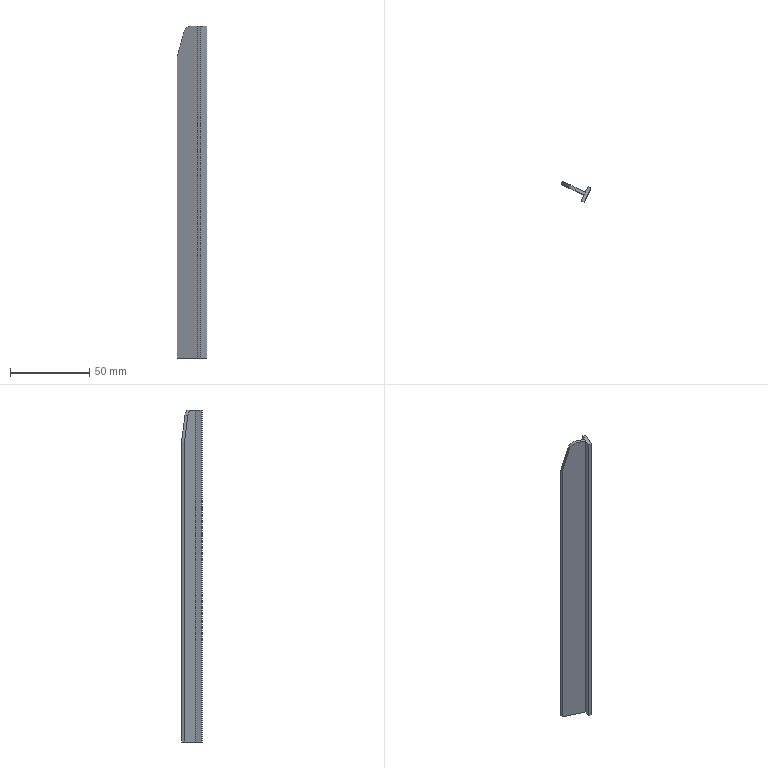Component | SolidWorks | JYTBJ-HeaderPlateClampBlock-1 | 1 solid | 12 faces | box 18.84 x 13.08 x 209 mm | volume 10743 mm3 | plane 11 | cylinder 1 | commonest cylinder face diameters 10 x1
build123d program:
from build123d import *

# Parameters (mm, degrees)
BOSS_EXTRUDE1_DEPTH = 209
CUT_EXTRUDE1_DEPTH  = 146
FILLET1_R           = 5


with BuildPart() as part:
    # Sketch1 → Boss-Extrude1 (new body)
    with BuildSketch(Plane.XY):
        Polygon((-5, 0), (5, 0), (5, 2), (1, 2), (1, 18), (-1, 18), (-1, 2), (-5, 2), align=None)
    extrude(amount=BOSS_EXTRUDE1_DEPTH)

    # Sketch3 → Cut-Extrude1 (cut)
    with BuildSketch(Plane(origin=(1, 0, 0), x_dir=(0, 0, -1), z_dir=(1, 0, 0))):
        Polygon((-20, 18), (0, 12), (0, 18), align=None)
    extrude(amount=-CUT_EXTRUDE1_DEPTH, mode=Mode.SUBTRACT)

    # Fillet1
    fillet1_edges = [part.edges().sort_by_distance(p)[0] for p in [
        (0, 12, 0),
    ]]
    fillet(fillet1_edges, radius=FILLET1_R)


solid = part.part

# Placed as in the assembly
solid = solid.moved(Location((-18.355, 107.069, 257.5), (-180, 0, 115.128)))
STEP:
#1=COLOUR_RGB('',0.7922,0.8196,0.9333);
#2=FILL_AREA_STYLE_COLOUR('',#1);
#3=FILL_AREA_STYLE('',(#2));
#4=SURFACE_STYLE_FILL_AREA(#3);
#5=SURFACE_SIDE_STYLE('',(#4));
#6=SURFACE_STYLE_USAGE(.BOTH.,#5);
#7=PRESENTATION_STYLE_ASSIGNMENT((#6));
#8=CARTESIAN_POINT('',(-1.348,4.552,9.35));
#9=VERTEX_POINT('',#8);
#10=CARTESIAN_POINT('',(-1.172,4.469,9.998));
#11=VERTEX_POINT('',#10);
#12=CARTESIAN_POINT('',(-3.155,5.399,2.697));
#13=DIRECTION('',(0.2602,-0.122,0.9578));
#14=VECTOR('',#13,39.37);
#15=LINE('',#12,#14);
#16=EDGE_CURVE('',#9,#11,#15,.T.);
#17=ORIENTED_EDGE('',*,*,#16,.T.);
#18=CARTESIAN_POINT('',(-1.001,4.389,10.138));
#19=VERTEX_POINT('',#18);
#20=CARTESIAN_POINT('',(-1.001,4.389,9.941));
#21=DIRECTION('',(0.4246,0.9054,0.));
#22=DIRECTION('',(0.,0.,1.));
#23=AXIS2_PLACEMENT_3D('',#20,#21,#22);
#24=CIRCLE('',#23,0.1969);
#25=EDGE_CURVE('',#11,#19,#24,.T.);
#26=ORIENTED_EDGE('',*,*,#25,.T.);
#27=CARTESIAN_POINT('',(-0.7772,4.284,10.138));
#28=VERTEX_POINT('',#27);
#29=CARTESIAN_POINT('',(-0.7772,4.284,10.138));
#30=DIRECTION('',(0.9054,-0.4246,0.));
#31=VECTOR('',#30,39.37);
#32=LINE('',#29,#31);
#33=EDGE_CURVE('',#19,#28,#32,.T.);
#34=ORIENTED_EDGE('',*,*,#33,.T.);
#35=CARTESIAN_POINT('',(-0.7772,4.284,1.909));
#36=VERTEX_POINT('',#35);
#37=CARTESIAN_POINT('',(-0.7772,4.284,1.909));
#38=DIRECTION('',(-0.,-0.,1.));
#39=VECTOR('',#38,39.37);
#40=LINE('',#37,#39);
#41=EDGE_CURVE('',#36,#28,#40,.T.);
#42=ORIENTED_EDGE('',*,*,#41,.F.);
#43=CARTESIAN_POINT('',(-1.348,4.552,1.909));
#44=VERTEX_POINT('',#43);
#45=CARTESIAN_POINT('',(-0.7772,4.284,1.909));
#46=DIRECTION('',(0.9054,-0.4246,0.));
#47=VECTOR('',#46,39.37);
#48=LINE('',#45,#47);
#49=EDGE_CURVE('',#44,#36,#48,.T.);
#50=ORIENTED_EDGE('',*,*,#49,.F.);
#51=CARTESIAN_POINT('',(-1.348,4.552,1.909));
#52=DIRECTION('',(-0.,-0.,1.));
#53=VECTOR('',#52,39.37);
#54=LINE('',#51,#53);
#55=EDGE_CURVE('',#44,#9,#54,.T.);
#56=ORIENTED_EDGE('',*,*,#55,.T.);
#57=EDGE_LOOP('',(#17,#26,#34,#42,#50,#56));
#58=FACE_OUTER_BOUND('',#57,.T.);
#59=CARTESIAN_POINT('',(-0.7772,4.284,1.909));
#60=DIRECTION('',(-0.4246,-0.9054,-0.));
#61=DIRECTION('',(-0.,-0.,1.));
#62=AXIS2_PLACEMENT_3D('',#59,#60,#61);
#63=PLANE('',#62);
#64=ADVANCED_FACE('',(#58),#63,.F.);
#65=CARTESIAN_POINT('',(-0.7104,4.427,10.138));
#66=VERTEX_POINT('',#65);
#67=CARTESIAN_POINT('',(-0.7104,4.427,10.138));
#68=DIRECTION('',(0.4246,0.9054,0.));
#69=VECTOR('',#68,39.37);
#70=LINE('',#67,#69);
#71=EDGE_CURVE('',#28,#66,#70,.T.);
#72=ORIENTED_EDGE('',*,*,#71,.T.);
#73=CARTESIAN_POINT('',(-0.7104,4.427,1.909));
#74=VERTEX_POINT('',#73);
#75=CARTESIAN_POINT('',(-0.7104,4.427,1.909));
#76=DIRECTION('',(-0.,-0.,1.));
#77=VECTOR('',#76,39.37);
#78=LINE('',#75,#77);
#79=EDGE_CURVE('',#74,#66,#78,.T.);
#80=ORIENTED_EDGE('',*,*,#79,.F.);
#81=CARTESIAN_POINT('',(-0.7104,4.427,1.909));
#82=DIRECTION('',(0.4246,0.9054,0.));
#83=VECTOR('',#82,39.37);
#84=LINE('',#81,#83);
#85=EDGE_CURVE('',#36,#74,#84,.T.);
#86=ORIENTED_EDGE('',*,*,#85,.F.);
#87=ORIENTED_EDGE('',*,*,#41,.T.);
#88=EDGE_LOOP('',(#72,#80,#86,#87));
#89=FACE_OUTER_BOUND('',#88,.T.);
#90=CARTESIAN_POINT('',(-0.7104,4.427,1.909));
#91=DIRECTION('',(0.9054,-0.4246,0.));
#92=DIRECTION('',(-0.4246,-0.9054,-0.));
#93=AXIS2_PLACEMENT_3D('',#90,#91,#92);
#94=PLANE('',#93);
#95=ADVANCED_FACE('',(#89),#94,.F.);
#96=CARTESIAN_POINT('',(-0.6391,4.394,10.138));
#97=VERTEX_POINT('',#96);
#98=CARTESIAN_POINT('',(-0.6391,4.394,10.138));
#99=DIRECTION('',(0.9054,-0.4246,0.));
#100=VECTOR('',#99,39.37);
#101=LINE('',#98,#100);
#102=EDGE_CURVE('',#66,#97,#101,.T.);
#103=ORIENTED_EDGE('',*,*,#102,.T.);
#104=CARTESIAN_POINT('',(-0.6391,4.394,1.909));
#105=VERTEX_POINT('',#104);
#106=CARTESIAN_POINT('',(-0.6391,4.394,1.909));
#107=DIRECTION('',(-0.,-0.,1.));
#108=VECTOR('',#107,39.37);
#109=LINE('',#106,#108);
#110=EDGE_CURVE('',#105,#97,#109,.T.);
#111=ORIENTED_EDGE('',*,*,#110,.F.);
#112=CARTESIAN_POINT('',(-0.6391,4.394,1.909));
#113=DIRECTION('',(0.9054,-0.4246,0.));
#114=VECTOR('',#113,39.37);
#115=LINE('',#112,#114);
#116=EDGE_CURVE('',#74,#105,#115,.T.);
#117=ORIENTED_EDGE('',*,*,#116,.F.);
#118=ORIENTED_EDGE('',*,*,#79,.T.);
#119=EDGE_LOOP('',(#103,#111,#117,#118));
#120=FACE_OUTER_BOUND('',#119,.T.);
#121=CARTESIAN_POINT('',(-0.6391,4.394,1.909));
#122=DIRECTION('',(-0.4246,-0.9054,-0.));
#123=DIRECTION('',(-0.,-0.,1.));
#124=AXIS2_PLACEMENT_3D('',#121,#122,#123);
#125=PLANE('',#124);
#126=ADVANCED_FACE('',(#120),#125,.F.);
#127=CARTESIAN_POINT('',(-0.8062,4.037,10.138));
#128=VERTEX_POINT('',#127);
#129=CARTESIAN_POINT('',(-0.6391,4.394,10.138));
#130=DIRECTION('',(-0.4246,-0.9054,-0.));
#131=VECTOR('',#130,39.37);
#132=LINE('',#129,#131);
#133=EDGE_CURVE('',#97,#128,#132,.T.);
#134=ORIENTED_EDGE('',*,*,#133,.T.);
#135=CARTESIAN_POINT('',(-0.8062,4.037,1.909));
#136=VERTEX_POINT('',#135);
#137=CARTESIAN_POINT('',(-0.8062,4.037,1.909));
#138=DIRECTION('',(-0.,-0.,1.));
#139=VECTOR('',#138,39.37);
#140=LINE('',#137,#139);
#141=EDGE_CURVE('',#136,#128,#140,.T.);
#142=ORIENTED_EDGE('',*,*,#141,.F.);
#143=CARTESIAN_POINT('',(-0.6391,4.394,1.909));
#144=DIRECTION('',(-0.4246,-0.9054,-0.));
#145=VECTOR('',#144,39.37);
#146=LINE('',#143,#145);
#147=EDGE_CURVE('',#105,#136,#146,.T.);
#148=ORIENTED_EDGE('',*,*,#147,.F.);
#149=ORIENTED_EDGE('',*,*,#110,.T.);
#150=EDGE_LOOP('',(#134,#142,#148,#149));
#151=FACE_OUTER_BOUND('',#150,.T.);
#152=CARTESIAN_POINT('',(-0.6391,4.394,1.909));
#153=DIRECTION('',(-0.9054,0.4246,-0.));
#154=DIRECTION('',(0.,0.,-1.));
#155=AXIS2_PLACEMENT_3D('',#152,#153,#154);
#156=PLANE('',#155);
#157=ADVANCED_FACE('',(#151),#156,.F.);
#158=CARTESIAN_POINT('',(-0.8775,4.071,10.138));
#159=VERTEX_POINT('',#158);
#160=CARTESIAN_POINT('',(-0.8062,4.037,10.138));
#161=DIRECTION('',(-0.9054,0.4246,-0.));
#162=VECTOR('',#161,39.37);
#163=LINE('',#160,#162);
#164=EDGE_CURVE('',#128,#159,#163,.T.);
#165=ORIENTED_EDGE('',*,*,#164,.T.);
#166=CARTESIAN_POINT('',(-0.8775,4.071,1.909));
#167=VERTEX_POINT('',#166);
#168=CARTESIAN_POINT('',(-0.8775,4.071,1.909));
#169=DIRECTION('',(-0.,-0.,1.));
#170=VECTOR('',#169,39.37);
#171=LINE('',#168,#170);
#172=EDGE_CURVE('',#167,#159,#171,.T.);
#173=ORIENTED_EDGE('',*,*,#172,.F.);
#174=CARTESIAN_POINT('',(-0.8062,4.037,1.909));
#175=DIRECTION('',(-0.9054,0.4246,-0.));
#176=VECTOR('',#175,39.37);
#177=LINE('',#174,#176);
#178=EDGE_CURVE('',#136,#167,#177,.T.);
#179=ORIENTED_EDGE('',*,*,#178,.F.);
#180=ORIENTED_EDGE('',*,*,#141,.T.);
#181=EDGE_LOOP('',(#165,#173,#179,#180));
#182=FACE_OUTER_BOUND('',#181,.T.);
#183=CARTESIAN_POINT('',(-0.8062,4.037,1.909));
#184=DIRECTION('',(0.4246,0.9054,0.));
#185=DIRECTION('',(0.,0.,-1.));
#186=AXIS2_PLACEMENT_3D('',#183,#184,#185);
#187=PLANE('',#186);
#188=ADVANCED_FACE('',(#182),#187,.F.);
#189=CARTESIAN_POINT('',(-0.8107,4.213,10.138));
#190=VERTEX_POINT('',#189);
#191=CARTESIAN_POINT('',(-0.8775,4.071,10.138));
#192=DIRECTION('',(0.4246,0.9054,0.));
#193=VECTOR('',#192,39.37);
#194=LINE('',#191,#193);
#195=EDGE_CURVE('',#159,#190,#194,.T.);
#196=ORIENTED_EDGE('',*,*,#195,.T.);
#197=CARTESIAN_POINT('',(-0.8107,4.213,1.909));
#198=VERTEX_POINT('',#197);
#199=CARTESIAN_POINT('',(-0.8107,4.213,1.909));
#200=DIRECTION('',(-0.,-0.,1.));
#201=VECTOR('',#200,39.37);
#202=LINE('',#199,#201);
#203=EDGE_CURVE('',#198,#190,#202,.T.);
#204=ORIENTED_EDGE('',*,*,#203,.F.);
#205=CARTESIAN_POINT('',(-0.8775,4.071,1.909));
#206=DIRECTION('',(0.4246,0.9054,0.));
#207=VECTOR('',#206,39.37);
#208=LINE('',#205,#207);
#209=EDGE_CURVE('',#167,#198,#208,.T.);
#210=ORIENTED_EDGE('',*,*,#209,.F.);
#211=ORIENTED_EDGE('',*,*,#172,.T.);
#212=EDGE_LOOP('',(#196,#204,#210,#211));
#213=FACE_OUTER_BOUND('',#212,.T.);
#214=CARTESIAN_POINT('',(-0.8775,4.071,1.909));
#215=DIRECTION('',(0.9054,-0.4246,0.));
#216=DIRECTION('',(-0.4246,-0.9054,-0.));
#217=AXIS2_PLACEMENT_3D('',#214,#215,#216);
#218=PLANE('',#217);
#219=ADVANCED_FACE('',(#213),#218,.F.);
#220=CARTESIAN_POINT('',(-1.034,4.318,10.138));
#221=VERTEX_POINT('',#220);
#222=CARTESIAN_POINT('',(-0.8107,4.213,10.138));
#223=DIRECTION('',(-0.9054,0.4246,-0.));
#224=VECTOR('',#223,39.37);
#225=LINE('',#222,#224);
#226=EDGE_CURVE('',#190,#221,#225,.T.);
#227=ORIENTED_EDGE('',*,*,#226,.T.);
#228=CARTESIAN_POINT('',(-1.205,4.398,9.998));
#229=VERTEX_POINT('',#228);
#230=CARTESIAN_POINT('',(-1.034,4.318,9.941));
#231=DIRECTION('',(-0.4246,-0.9054,-0.));
#232=DIRECTION('',(0.,0.,-1.));
#233=AXIS2_PLACEMENT_3D('',#230,#231,#232);
#234=CIRCLE('',#233,0.1969);
#235=EDGE_CURVE('',#221,#229,#234,.T.);
#236=ORIENTED_EDGE('',*,*,#235,.T.);
#237=CARTESIAN_POINT('',(-1.381,4.481,9.35));
#238=VERTEX_POINT('',#237);
#239=CARTESIAN_POINT('',(-1.381,4.481,9.35));
#240=DIRECTION('',(0.2602,-0.122,0.9578));
#241=VECTOR('',#240,39.37);
#242=LINE('',#239,#241);
#243=EDGE_CURVE('',#238,#229,#242,.T.);
#244=ORIENTED_EDGE('',*,*,#243,.F.);
#245=CARTESIAN_POINT('',(-1.381,4.481,1.909));
#246=VERTEX_POINT('',#245);
#247=CARTESIAN_POINT('',(-1.381,4.481,1.909));
#248=DIRECTION('',(-0.,-0.,1.));
#249=VECTOR('',#248,39.37);
#250=LINE('',#247,#249);
#251=EDGE_CURVE('',#246,#238,#250,.T.);
#252=ORIENTED_EDGE('',*,*,#251,.F.);
#253=CARTESIAN_POINT('',(-0.8107,4.213,1.909));
#254=DIRECTION('',(-0.9054,0.4246,-0.));
#255=VECTOR('',#254,39.37);
#256=LINE('',#253,#255);
#257=EDGE_CURVE('',#198,#246,#256,.T.);
#258=ORIENTED_EDGE('',*,*,#257,.F.);
#259=ORIENTED_EDGE('',*,*,#203,.T.);
#260=EDGE_LOOP('',(#227,#236,#244,#252,#258,#259));
#261=FACE_OUTER_BOUND('',#260,.T.);
#262=CARTESIAN_POINT('',(-0.8107,4.213,1.909));
#263=DIRECTION('',(0.4246,0.9054,0.));
#264=DIRECTION('',(0.,0.,-1.));
#265=AXIS2_PLACEMENT_3D('',#262,#263,#264);
#266=PLANE('',#265);
#267=ADVANCED_FACE('',(#261),#266,.F.);
#268=ORIENTED_EDGE('',*,*,#251,.T.);
#269=CARTESIAN_POINT('',(1.06,9.685,9.35));
#270=DIRECTION('',(-0.4246,-0.9054,-0.));
#271=VECTOR('',#270,39.37);
#272=LINE('',#269,#271);
#273=EDGE_CURVE('',#9,#238,#272,.T.);
#274=ORIENTED_EDGE('',*,*,#273,.F.);
#275=ORIENTED_EDGE('',*,*,#55,.F.);
#276=CARTESIAN_POINT('',(-1.381,4.481,1.909));
#277=DIRECTION('',(0.4246,0.9054,0.));
#278=VECTOR('',#277,39.37);
#279=LINE('',#276,#278);
#280=EDGE_CURVE('',#246,#44,#279,.T.);
#281=ORIENTED_EDGE('',*,*,#280,.F.);
#282=EDGE_LOOP('',(#268,#274,#275,#281));
#283=FACE_OUTER_BOUND('',#282,.T.);
#284=CARTESIAN_POINT('',(-1.381,4.481,1.909));
#285=DIRECTION('',(0.9054,-0.4246,0.));
#286=DIRECTION('',(-0.,-0.,1.));
#287=AXIS2_PLACEMENT_3D('',#284,#285,#286);
#288=PLANE('',#287);
#289=ADVANCED_FACE('',(#283),#288,.F.);
#290=ORIENTED_EDGE('',*,*,#49,.T.);
#291=ORIENTED_EDGE('',*,*,#85,.T.);
#292=ORIENTED_EDGE('',*,*,#116,.T.);
#293=ORIENTED_EDGE('',*,*,#147,.T.);
#294=ORIENTED_EDGE('',*,*,#178,.T.);
#295=ORIENTED_EDGE('',*,*,#209,.T.);
#296=ORIENTED_EDGE('',*,*,#257,.T.);
#297=ORIENTED_EDGE('',*,*,#280,.T.);
#298=EDGE_LOOP('',(#290,#291,#292,#293,#294,#295,#296,#297));
#299=FACE_OUTER_BOUND('',#298,.T.);
#300=CARTESIAN_POINT('',(-1.348,4.552,1.909));
#301=DIRECTION('',(0.,0.,-1.));
#302=DIRECTION('',(-0.4246,-0.9054,-0.));
#303=AXIS2_PLACEMENT_3D('',#300,#301,#302);
#304=PLANE('',#303);
#305=ADVANCED_FACE('',(#299),#304,.T.);
#306=ORIENTED_EDGE('',*,*,#33,.F.);
#307=CARTESIAN_POINT('',(-1.001,4.389,10.138));
#308=DIRECTION('',(-0.4246,-0.9054,-0.));
#309=VECTOR('',#308,39.37);
#310=LINE('',#307,#309);
#311=EDGE_CURVE('',#19,#221,#310,.T.);
#312=ORIENTED_EDGE('',*,*,#311,.T.);
#313=ORIENTED_EDGE('',*,*,#226,.F.);
#314=ORIENTED_EDGE('',*,*,#195,.F.);
#315=ORIENTED_EDGE('',*,*,#164,.F.);
#316=ORIENTED_EDGE('',*,*,#133,.F.);
#317=ORIENTED_EDGE('',*,*,#102,.F.);
#318=ORIENTED_EDGE('',*,*,#71,.F.);
#319=EDGE_LOOP('',(#306,#312,#313,#314,#315,#316,#317,#318));
#320=FACE_OUTER_BOUND('',#319,.T.);
#321=CARTESIAN_POINT('',(-1.348,4.552,10.138));
#322=DIRECTION('',(0.,0.,-1.));
#323=DIRECTION('',(-0.4246,-0.9054,-0.));
#324=AXIS2_PLACEMENT_3D('',#321,#322,#323);
#325=PLANE('',#324);
#326=ADVANCED_FACE('',(#320),#325,.F.);
#327=ORIENTED_EDGE('',*,*,#243,.T.);
#328=CARTESIAN_POINT('',(1.236,9.602,9.998));
#329=DIRECTION('',(0.4246,0.9054,0.));
#330=VECTOR('',#329,39.37);
#331=LINE('',#328,#330);
#332=EDGE_CURVE('',#229,#11,#331,.T.);
#333=ORIENTED_EDGE('',*,*,#332,.T.);
#334=ORIENTED_EDGE('',*,*,#16,.F.);
#335=ORIENTED_EDGE('',*,*,#273,.T.);
#336=EDGE_LOOP('',(#327,#333,#334,#335));
#337=FACE_OUTER_BOUND('',#336,.T.);
#338=CARTESIAN_POINT('',(1.06,9.685,9.35));
#339=DIRECTION('',(0.8672,-0.4067,-0.2873));
#340=DIRECTION('',(0.2602,-0.122,0.9578));
#341=AXIS2_PLACEMENT_3D('',#338,#339,#340);
#342=PLANE('',#341);
#343=ADVANCED_FACE('',(#337),#342,.F.);
#344=ORIENTED_EDGE('',*,*,#25,.F.);
#345=ORIENTED_EDGE('',*,*,#332,.F.);
#346=ORIENTED_EDGE('',*,*,#235,.F.);
#347=ORIENTED_EDGE('',*,*,#311,.F.);
#348=EDGE_LOOP('',(#344,#345,#346,#347));
#349=FACE_OUTER_BOUND('',#348,.T.);
#350=CARTESIAN_POINT('',(-1.001,4.389,9.941));
#351=DIRECTION('',(-0.4246,-0.9054,-0.));
#352=DIRECTION('',(0.,0.,1.));
#353=AXIS2_PLACEMENT_3D('',#350,#351,#352);
#354=CYLINDRICAL_SURFACE('',#353,0.1969);
#355=ADVANCED_FACE('',(#349),#354,.T.);
#356=CLOSED_SHELL('',(#64,#95,#126,#157,#188,#219,#267,#289,#305,#326,#343,#355));
#357=MANIFOLD_SOLID_BREP('',#356);
#358=STYLED_ITEM('',(#7),#357);
#359=PRESENTATION_LAYER_ASSIGNMENT('','',(#358));
#360=CARTESIAN_POINT('',(0.,0.,0.));
#361=DIRECTION('',(0.,0.,1.));
#362=DIRECTION('',(1.,0.,0.));
#363=AXIS2_PLACEMENT_3D('',#360,#361,#362);
#364=(LENGTH_UNIT()NAMED_UNIT(*)SI_UNIT($,.METRE.));
#365=LENGTH_MEASURE_WITH_UNIT(LENGTH_MEASURE(0.0254),#364);
#366=DIMENSIONAL_EXPONENTS(1.,0.,0.,0.,0.,0.,0.);
#367=(CONVERSION_BASED_UNIT('',#365)LENGTH_UNIT()NAMED_UNIT(#366));
#368=UNCERTAINTY_MEASURE_WITH_UNIT(LENGTH_MEASURE(0.00001),#367,'','');
#369=(NAMED_UNIT(*)PLANE_ANGLE_UNIT()SI_UNIT($,.RADIAN.));
#370=(NAMED_UNIT(*)SI_UNIT($,.STERADIAN.)SOLID_ANGLE_UNIT());
#371=(GEOMETRIC_REPRESENTATION_CONTEXT(3)GLOBAL_UNCERTAINTY_ASSIGNED_CONTEXT((#368))GLOBAL_UNIT_ASSIGNED_CONTEXT((#367,#369,#370))REPRESENTATION_CONTEXT('',''));
#372=ADVANCED_BREP_SHAPE_REPRESENTATION('',(#357,#363),#371);
#373=(LENGTH_UNIT()NAMED_UNIT(*)SI_UNIT($,.METRE.));
#374=LENGTH_MEASURE_WITH_UNIT(LENGTH_MEASURE(0.0254),#373);
#375=DIMENSIONAL_EXPONENTS(1.,0.,0.,0.,0.,0.,0.);
#376=(CONVERSION_BASED_UNIT('',#374)LENGTH_UNIT()NAMED_UNIT(#375));
#377=UNCERTAINTY_MEASURE_WITH_UNIT(LENGTH_MEASURE(0.00001),#376,'','');
#378=(NAMED_UNIT(*)PLANE_ANGLE_UNIT()SI_UNIT($,.RADIAN.));
#379=(NAMED_UNIT(*)SI_UNIT($,.STERADIAN.)SOLID_ANGLE_UNIT());
#380=(GEOMETRIC_REPRESENTATION_CONTEXT(3)GLOBAL_UNCERTAINTY_ASSIGNED_CONTEXT((#377))GLOBAL_UNIT_ASSIGNED_CONTEXT((#376,#378,#379))REPRESENTATION_CONTEXT('',''));
#381=MECHANICAL_DESIGN_GEOMETRIC_PRESENTATION_REPRESENTATION('',(#358),#380);